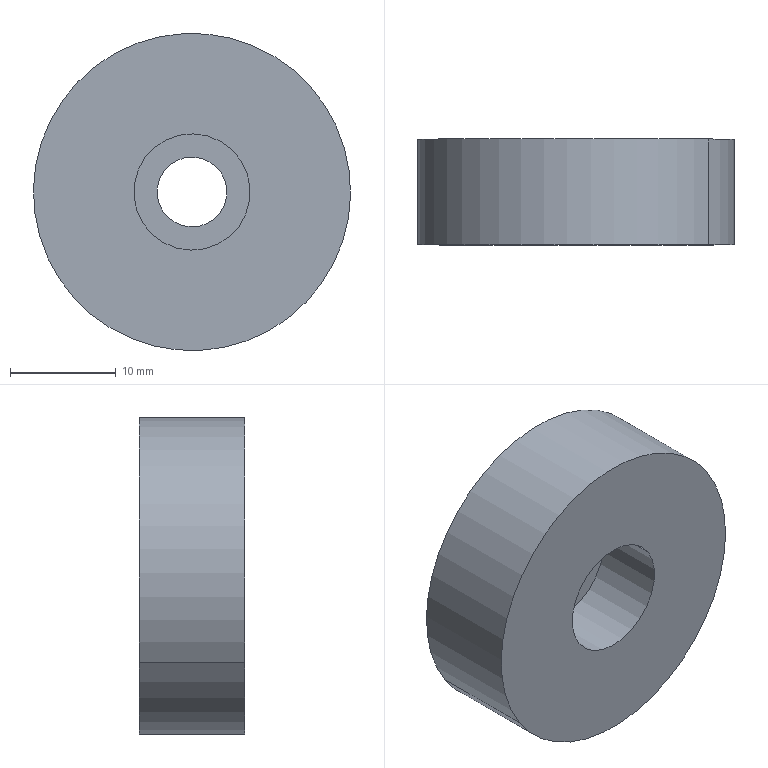Component | SolidWorks | JL001-05-03-1_JL001-05-01-009-1 | 1 solid | 9 faces | box 30 x 10 x 30 mm | volume 6313 mm3 | cylinder 6 | plane 3 | commonest cylinder face diameters 11 x2 6.6 x2 30 x2
build123d program:
from build123d import *

# Parameters (mm, degrees)
SKETCH1_R                                         = 15
BOSS_EXTRUDE1_DEPTH                               = 10
HOLE_SIZE_ACCORDING_TO_TYPE_1_OF_HEXA_D           = 6.6
HOLE_SIZE_ACCORDING_TO_TYPE_1_OF_HEXA_CBORE_D     = 11
HOLE_SIZE_ACCORDING_TO_TYPE_1_OF_HEXA_CBORE_DEPTH = 6.8


with BuildPart() as part:
    # Sketch1 → Boss-Extrude1 (new body)
    with BuildSketch(Plane(origin=(0, 0, 0), x_dir=(1, 0, 0), z_dir=(0, 1, 0))):
        with Locations(Location((0, 0, 0), (0, 0, 270))):
            Circle(SKETCH1_R)
    extrude(amount=BOSS_EXTRUDE1_DEPTH)

    # Hole Size _ according to_ Type 1 of Hexa (through all)
    with Locations(Plane(origin=(0, 10, 0), x_dir=(1, 0, 0), z_dir=(0, 1, 0))):
        with Locations((0, 0)):
            CounterBoreHole(HOLE_SIZE_ACCORDING_TO_TYPE_1_OF_HEXA_D / 2, HOLE_SIZE_ACCORDING_TO_TYPE_1_OF_HEXA_CBORE_D / 2, HOLE_SIZE_ACCORDING_TO_TYPE_1_OF_HEXA_CBORE_DEPTH)


solid = part.part

# Placed as in the assembly
solid = solid.moved(Location((0, 232.348, 63), (180, 0, 0)))
STEP:
#1=COLOUR_RGB('',0.7922,0.8196,0.9333);
#2=FILL_AREA_STYLE_COLOUR('',#1);
#3=FILL_AREA_STYLE('',(#2));
#4=SURFACE_STYLE_FILL_AREA(#3);
#5=SURFACE_SIDE_STYLE('',(#4));
#6=SURFACE_STYLE_USAGE(.BOTH.,#5);
#7=PRESENTATION_STYLE_ASSIGNMENT((#6));
#8=CARTESIAN_POINT('',(-0.1813,9.022,2.362));
#9=VERTEX_POINT('',#8);
#10=CARTESIAN_POINT('',(0.1813,9.022,2.599));
#11=VERTEX_POINT('',#10);
#12=CARTESIAN_POINT('',(-0.,9.022,2.48));
#13=DIRECTION('',(0.,-1.,0.));
#14=DIRECTION('',(0.8372,0.,0.5469));
#15=AXIS2_PLACEMENT_3D('',#12,#13,#14);
#16=CIRCLE('',#15,0.2165);
#17=EDGE_CURVE('',#9,#11,#16,.T.);
#18=ORIENTED_EDGE('',*,*,#17,.F.);
#19=CARTESIAN_POINT('',(-0.1813,8.754,2.362));
#20=VERTEX_POINT('',#19);
#21=CARTESIAN_POINT('',(-0.1813,8.754,2.362));
#22=DIRECTION('',(0.,-1.,0.));
#23=VECTOR('',#22,39.37);
#24=LINE('',#21,#23);
#25=EDGE_CURVE('',#9,#20,#24,.T.);
#26=ORIENTED_EDGE('',*,*,#25,.T.);
#27=CARTESIAN_POINT('',(0.1813,8.754,2.599));
#28=VERTEX_POINT('',#27);
#29=CARTESIAN_POINT('',(-0.,8.754,2.48));
#30=DIRECTION('',(0.,-1.,0.));
#31=DIRECTION('',(0.8372,0.,0.5469));
#32=AXIS2_PLACEMENT_3D('',#29,#30,#31);
#33=CIRCLE('',#32,0.2165);
#34=EDGE_CURVE('',#20,#28,#33,.T.);
#35=ORIENTED_EDGE('',*,*,#34,.T.);
#36=CARTESIAN_POINT('',(0.1813,8.754,2.599));
#37=DIRECTION('',(0.,-1.,0.));
#38=VECTOR('',#37,39.37);
#39=LINE('',#36,#38);
#40=EDGE_CURVE('',#11,#28,#39,.T.);
#41=ORIENTED_EDGE('',*,*,#40,.F.);
#42=EDGE_LOOP('',(#18,#26,#35,#41));
#43=FACE_OUTER_BOUND('',#42,.T.);
#44=CARTESIAN_POINT('',(-0.,8.754,2.48));
#45=DIRECTION('',(0.,-1.,0.));
#46=DIRECTION('',(0.8372,0.,0.5469));
#47=AXIS2_PLACEMENT_3D('',#44,#45,#46);
#48=CYLINDRICAL_SURFACE('',#47,0.2165);
#49=ADVANCED_FACE('',(#43),#48,.F.);
#50=CARTESIAN_POINT('',(-0.1088,9.148,2.409));
#51=VERTEX_POINT('',#50);
#52=CARTESIAN_POINT('',(0.1088,9.148,2.551));
#53=VERTEX_POINT('',#52);
#54=CARTESIAN_POINT('',(-0.,9.148,2.48));
#55=DIRECTION('',(0.,-1.,0.));
#56=DIRECTION('',(0.8372,0.,0.5469));
#57=AXIS2_PLACEMENT_3D('',#54,#55,#56);
#58=CIRCLE('',#57,0.1299);
#59=EDGE_CURVE('',#51,#53,#58,.T.);
#60=ORIENTED_EDGE('',*,*,#59,.F.);
#61=CARTESIAN_POINT('',(-0.1088,9.022,2.409));
#62=VERTEX_POINT('',#61);
#63=CARTESIAN_POINT('',(-0.1088,8.754,2.409));
#64=DIRECTION('',(0.,-1.,0.));
#65=VECTOR('',#64,39.37);
#66=LINE('',#63,#65);
#67=EDGE_CURVE('',#51,#62,#66,.T.);
#68=ORIENTED_EDGE('',*,*,#67,.T.);
#69=CARTESIAN_POINT('',(0.1088,9.022,2.551));
#70=VERTEX_POINT('',#69);
#71=CARTESIAN_POINT('',(-0.,9.022,2.48));
#72=DIRECTION('',(0.,-1.,0.));
#73=DIRECTION('',(0.8372,0.,0.5469));
#74=AXIS2_PLACEMENT_3D('',#71,#72,#73);
#75=CIRCLE('',#74,0.1299);
#76=EDGE_CURVE('',#62,#70,#75,.T.);
#77=ORIENTED_EDGE('',*,*,#76,.T.);
#78=CARTESIAN_POINT('',(0.1088,8.754,2.551));
#79=DIRECTION('',(0.,-1.,0.));
#80=VECTOR('',#79,39.37);
#81=LINE('',#78,#80);
#82=EDGE_CURVE('',#53,#70,#81,.T.);
#83=ORIENTED_EDGE('',*,*,#82,.F.);
#84=EDGE_LOOP('',(#60,#68,#77,#83));
#85=FACE_OUTER_BOUND('',#84,.T.);
#86=CARTESIAN_POINT('',(-0.,8.754,2.48));
#87=DIRECTION('',(0.,-1.,0.));
#88=DIRECTION('',(0.8372,0.,0.5469));
#89=AXIS2_PLACEMENT_3D('',#86,#87,#88);
#90=CYLINDRICAL_SURFACE('',#89,0.1299);
#91=ADVANCED_FACE('',(#85),#90,.F.);
#92=CARTESIAN_POINT('',(0.4944,8.754,2.803));
#93=VERTEX_POINT('',#92);
#94=CARTESIAN_POINT('',(-0.4944,8.754,2.157));
#95=VERTEX_POINT('',#94);
#96=CARTESIAN_POINT('',(-0.,8.754,2.48));
#97=DIRECTION('',(0.,-1.,0.));
#98=DIRECTION('',(0.8372,0.,0.5469));
#99=AXIS2_PLACEMENT_3D('',#96,#97,#98);
#100=CIRCLE('',#99,0.5906);
#101=EDGE_CURVE('',#93,#95,#100,.T.);
#102=ORIENTED_EDGE('',*,*,#101,.F.);
#103=CARTESIAN_POINT('',(0.4944,9.148,2.803));
#104=VERTEX_POINT('',#103);
#105=CARTESIAN_POINT('',(0.4944,8.754,2.803));
#106=DIRECTION('',(0.,1.,0.));
#107=VECTOR('',#106,39.37);
#108=LINE('',#105,#107);
#109=EDGE_CURVE('',#93,#104,#108,.T.);
#110=ORIENTED_EDGE('',*,*,#109,.T.);
#111=CARTESIAN_POINT('',(-0.4944,9.148,2.157));
#112=VERTEX_POINT('',#111);
#113=CARTESIAN_POINT('',(-0.,9.148,2.48));
#114=DIRECTION('',(0.,-1.,0.));
#115=DIRECTION('',(0.8372,0.,0.5469));
#116=AXIS2_PLACEMENT_3D('',#113,#114,#115);
#117=CIRCLE('',#116,0.5906);
#118=EDGE_CURVE('',#104,#112,#117,.T.);
#119=ORIENTED_EDGE('',*,*,#118,.T.);
#120=CARTESIAN_POINT('',(-0.4944,8.754,2.157));
#121=DIRECTION('',(0.,1.,0.));
#122=VECTOR('',#121,39.37);
#123=LINE('',#120,#122);
#124=EDGE_CURVE('',#95,#112,#123,.T.);
#125=ORIENTED_EDGE('',*,*,#124,.F.);
#126=EDGE_LOOP('',(#102,#110,#119,#125));
#127=FACE_OUTER_BOUND('',#126,.T.);
#128=CARTESIAN_POINT('',(-0.,8.754,2.48));
#129=DIRECTION('',(0.,1.,0.));
#130=DIRECTION('',(-0.8372,0.,-0.5469));
#131=AXIS2_PLACEMENT_3D('',#128,#129,#130);
#132=CYLINDRICAL_SURFACE('',#131,0.5906);
#133=ADVANCED_FACE('',(#127),#132,.T.);
#134=ORIENTED_EDGE('',*,*,#109,.F.);
#135=CARTESIAN_POINT('',(-0.,8.754,2.48));
#136=DIRECTION('',(0.,-1.,0.));
#137=DIRECTION('',(0.8372,0.,0.5469));
#138=AXIS2_PLACEMENT_3D('',#135,#136,#137);
#139=CIRCLE('',#138,0.5906);
#140=EDGE_CURVE('',#95,#93,#139,.T.);
#141=ORIENTED_EDGE('',*,*,#140,.F.);
#142=ORIENTED_EDGE('',*,*,#124,.T.);
#143=CARTESIAN_POINT('',(-0.,9.148,2.48));
#144=DIRECTION('',(0.,-1.,0.));
#145=DIRECTION('',(0.8372,0.,0.5469));
#146=AXIS2_PLACEMENT_3D('',#143,#144,#145);
#147=CIRCLE('',#146,0.5906);
#148=EDGE_CURVE('',#112,#104,#147,.T.);
#149=ORIENTED_EDGE('',*,*,#148,.T.);
#150=EDGE_LOOP('',(#134,#141,#142,#149));
#151=FACE_OUTER_BOUND('',#150,.T.);
#152=CARTESIAN_POINT('',(-0.,8.754,2.48));
#153=DIRECTION('',(0.,1.,0.));
#154=DIRECTION('',(-0.8372,0.,-0.5469));
#155=AXIS2_PLACEMENT_3D('',#152,#153,#154);
#156=CYLINDRICAL_SURFACE('',#155,0.5906);
#157=ADVANCED_FACE('',(#151),#156,.T.);
#158=CARTESIAN_POINT('',(-0.,8.754,2.48));
#159=DIRECTION('',(0.,-1.,0.));
#160=DIRECTION('',(0.8372,0.,0.5469));
#161=AXIS2_PLACEMENT_3D('',#158,#159,#160);
#162=CIRCLE('',#161,0.2165);
#163=EDGE_CURVE('',#28,#20,#162,.T.);
#164=ORIENTED_EDGE('',*,*,#163,.F.);
#165=ORIENTED_EDGE('',*,*,#34,.F.);
#166=EDGE_LOOP('',(#164,#165));
#167=FACE_BOUND('',#166,.T.);
#168=ORIENTED_EDGE('',*,*,#140,.T.);
#169=ORIENTED_EDGE('',*,*,#101,.T.);
#170=EDGE_LOOP('',(#168,#169));
#171=FACE_OUTER_BOUND('',#170,.T.);
#172=CARTESIAN_POINT('',(-0.,8.754,2.48));
#173=DIRECTION('',(0.,-1.,0.));
#174=DIRECTION('',(0.8372,0.,0.5469));
#175=AXIS2_PLACEMENT_3D('',#172,#173,#174);
#176=PLANE('',#175);
#177=ADVANCED_FACE('',(#167,#171),#176,.T.);
#178=CARTESIAN_POINT('',(-0.,9.148,2.48));
#179=DIRECTION('',(0.,-1.,0.));
#180=DIRECTION('',(0.8372,0.,0.5469));
#181=AXIS2_PLACEMENT_3D('',#178,#179,#180);
#182=CIRCLE('',#181,0.1299);
#183=EDGE_CURVE('',#53,#51,#182,.T.);
#184=ORIENTED_EDGE('',*,*,#183,.T.);
#185=ORIENTED_EDGE('',*,*,#59,.T.);
#186=EDGE_LOOP('',(#184,#185));
#187=FACE_BOUND('',#186,.T.);
#188=ORIENTED_EDGE('',*,*,#148,.F.);
#189=ORIENTED_EDGE('',*,*,#118,.F.);
#190=EDGE_LOOP('',(#188,#189));
#191=FACE_OUTER_BOUND('',#190,.T.);
#192=CARTESIAN_POINT('',(-0.,9.148,2.48));
#193=DIRECTION('',(0.,-1.,0.));
#194=DIRECTION('',(0.8372,0.,0.5469));
#195=AXIS2_PLACEMENT_3D('',#192,#193,#194);
#196=PLANE('',#195);
#197=ADVANCED_FACE('',(#187,#191),#196,.F.);
#198=ORIENTED_EDGE('',*,*,#67,.F.);
#199=ORIENTED_EDGE('',*,*,#183,.F.);
#200=ORIENTED_EDGE('',*,*,#82,.T.);
#201=CARTESIAN_POINT('',(-0.,9.022,2.48));
#202=DIRECTION('',(0.,-1.,0.));
#203=DIRECTION('',(0.8372,0.,0.5469));
#204=AXIS2_PLACEMENT_3D('',#201,#202,#203);
#205=CIRCLE('',#204,0.1299);
#206=EDGE_CURVE('',#70,#62,#205,.T.);
#207=ORIENTED_EDGE('',*,*,#206,.T.);
#208=EDGE_LOOP('',(#198,#199,#200,#207));
#209=FACE_OUTER_BOUND('',#208,.T.);
#210=CARTESIAN_POINT('',(-0.,8.754,2.48));
#211=DIRECTION('',(0.,-1.,0.));
#212=DIRECTION('',(0.8372,0.,0.5469));
#213=AXIS2_PLACEMENT_3D('',#210,#211,#212);
#214=CYLINDRICAL_SURFACE('',#213,0.1299);
#215=ADVANCED_FACE('',(#209),#214,.F.);
#216=ORIENTED_EDGE('',*,*,#206,.F.);
#217=ORIENTED_EDGE('',*,*,#76,.F.);
#218=EDGE_LOOP('',(#216,#217));
#219=FACE_BOUND('',#218,.T.);
#220=CARTESIAN_POINT('',(-0.,9.022,2.48));
#221=DIRECTION('',(0.,-1.,0.));
#222=DIRECTION('',(0.8372,0.,0.5469));
#223=AXIS2_PLACEMENT_3D('',#220,#221,#222);
#224=CIRCLE('',#223,0.2165);
#225=EDGE_CURVE('',#11,#9,#224,.T.);
#226=ORIENTED_EDGE('',*,*,#225,.T.);
#227=ORIENTED_EDGE('',*,*,#17,.T.);
#228=EDGE_LOOP('',(#226,#227));
#229=FACE_OUTER_BOUND('',#228,.T.);
#230=CARTESIAN_POINT('',(-0.07106,9.022,2.589));
#231=DIRECTION('',(0.,1.,0.));
#232=DIRECTION('',(-0.8372,0.,-0.5469));
#233=AXIS2_PLACEMENT_3D('',#230,#231,#232);
#234=PLANE('',#233);
#235=ADVANCED_FACE('',(#219,#229),#234,.F.);
#236=ORIENTED_EDGE('',*,*,#25,.F.);
#237=ORIENTED_EDGE('',*,*,#225,.F.);
#238=ORIENTED_EDGE('',*,*,#40,.T.);
#239=ORIENTED_EDGE('',*,*,#163,.T.);
#240=EDGE_LOOP('',(#236,#237,#238,#239));
#241=FACE_OUTER_BOUND('',#240,.T.);
#242=CARTESIAN_POINT('',(-0.,8.754,2.48));
#243=DIRECTION('',(0.,-1.,0.));
#244=DIRECTION('',(0.8372,0.,0.5469));
#245=AXIS2_PLACEMENT_3D('',#242,#243,#244);
#246=CYLINDRICAL_SURFACE('',#245,0.2165);
#247=ADVANCED_FACE('',(#241),#246,.F.);
#248=CLOSED_SHELL('',(#49,#91,#133,#157,#177,#197,#215,#235,#247));
#249=MANIFOLD_SOLID_BREP('',#248);
#250=STYLED_ITEM('',(#7),#249);
#251=(LENGTH_UNIT()NAMED_UNIT(*)SI_UNIT($,.METRE.));
#252=LENGTH_MEASURE_WITH_UNIT(LENGTH_MEASURE(0.0254),#251);
#253=DIMENSIONAL_EXPONENTS(1.,0.,0.,0.,0.,0.,0.);
#254=(CONVERSION_BASED_UNIT('',#252)LENGTH_UNIT()NAMED_UNIT(#253));
#255=UNCERTAINTY_MEASURE_WITH_UNIT(LENGTH_MEASURE(0.00001),#254,'','');
#256=(NAMED_UNIT(*)PLANE_ANGLE_UNIT()SI_UNIT($,.RADIAN.));
#257=(NAMED_UNIT(*)SI_UNIT($,.STERADIAN.)SOLID_ANGLE_UNIT());
#258=(GEOMETRIC_REPRESENTATION_CONTEXT(3)GLOBAL_UNCERTAINTY_ASSIGNED_CONTEXT((#255))GLOBAL_UNIT_ASSIGNED_CONTEXT((#254,#256,#257))REPRESENTATION_CONTEXT('',''));
#259=MECHANICAL_DESIGN_GEOMETRIC_PRESENTATION_REPRESENTATION('',(#250),#258);
#260=PRESENTATION_LAYER_ASSIGNMENT('','',(#250));
#261=CARTESIAN_POINT('',(0.,0.,0.));
#262=DIRECTION('',(0.,0.,1.));
#263=DIRECTION('',(1.,0.,0.));
#264=AXIS2_PLACEMENT_3D('',#261,#262,#263);
#265=(LENGTH_UNIT()NAMED_UNIT(*)SI_UNIT($,.METRE.));
#266=LENGTH_MEASURE_WITH_UNIT(LENGTH_MEASURE(0.0254),#265);
#267=DIMENSIONAL_EXPONENTS(1.,0.,0.,0.,0.,0.,0.);
#268=(CONVERSION_BASED_UNIT('',#266)LENGTH_UNIT()NAMED_UNIT(#267));
#269=UNCERTAINTY_MEASURE_WITH_UNIT(LENGTH_MEASURE(0.00001),#268,'','');
#270=(NAMED_UNIT(*)PLANE_ANGLE_UNIT()SI_UNIT($,.RADIAN.));
#271=(NAMED_UNIT(*)SI_UNIT($,.STERADIAN.)SOLID_ANGLE_UNIT());
#272=(GEOMETRIC_REPRESENTATION_CONTEXT(3)GLOBAL_UNCERTAINTY_ASSIGNED_CONTEXT((#269))GLOBAL_UNIT_ASSIGNED_CONTEXT((#268,#270,#271))REPRESENTATION_CONTEXT('',''));
#273=ADVANCED_BREP_SHAPE_REPRESENTATION('',(#249,#264),#272);